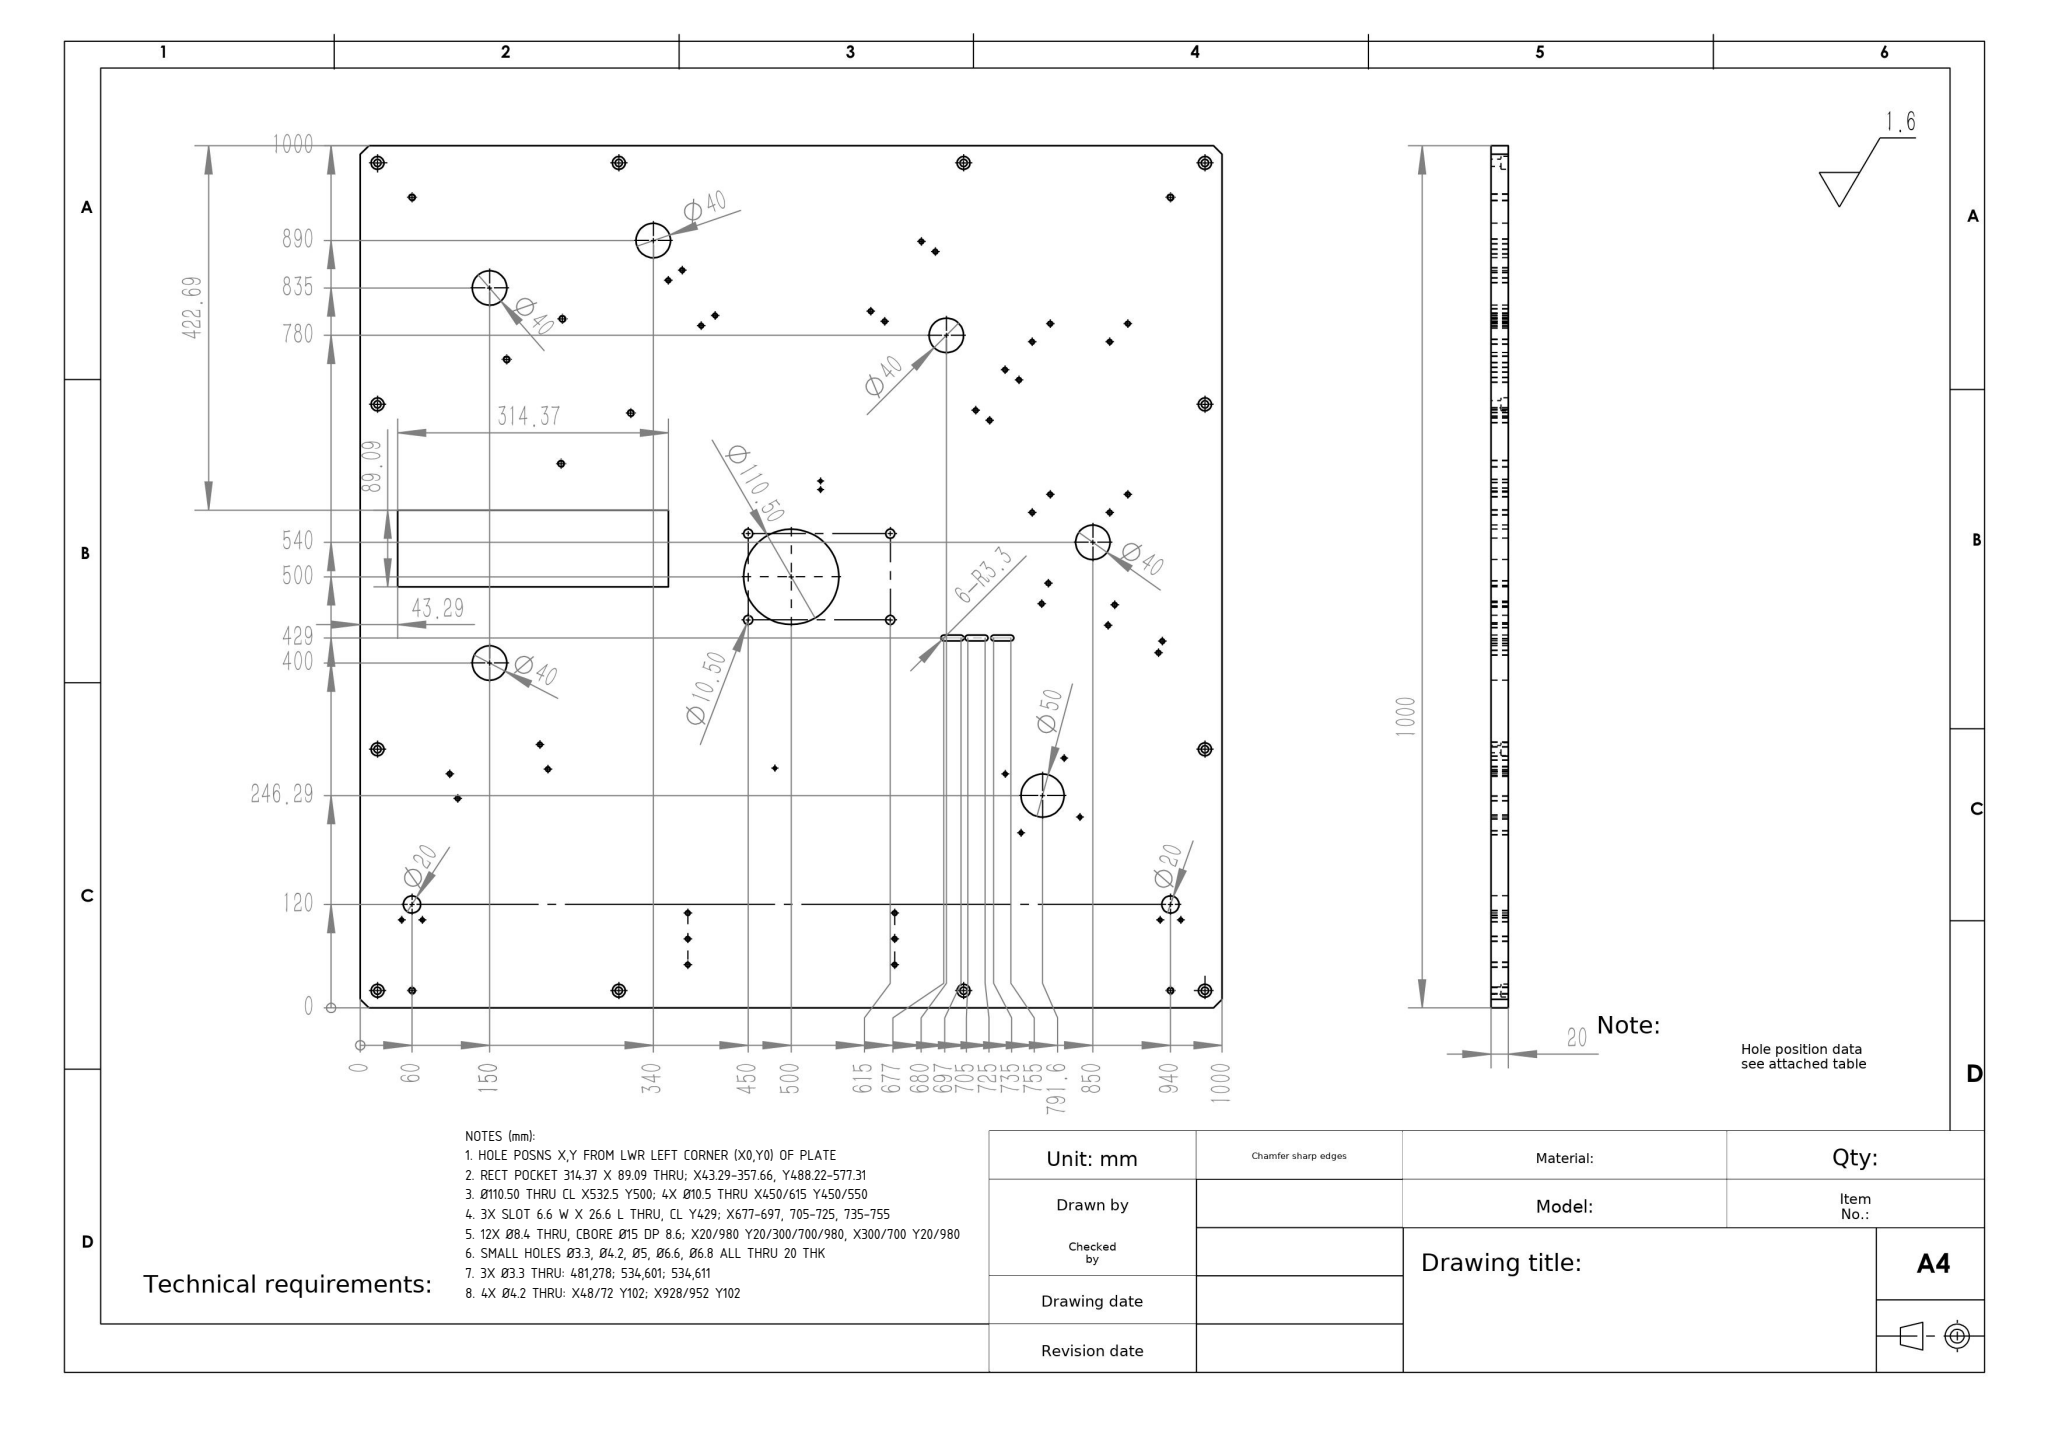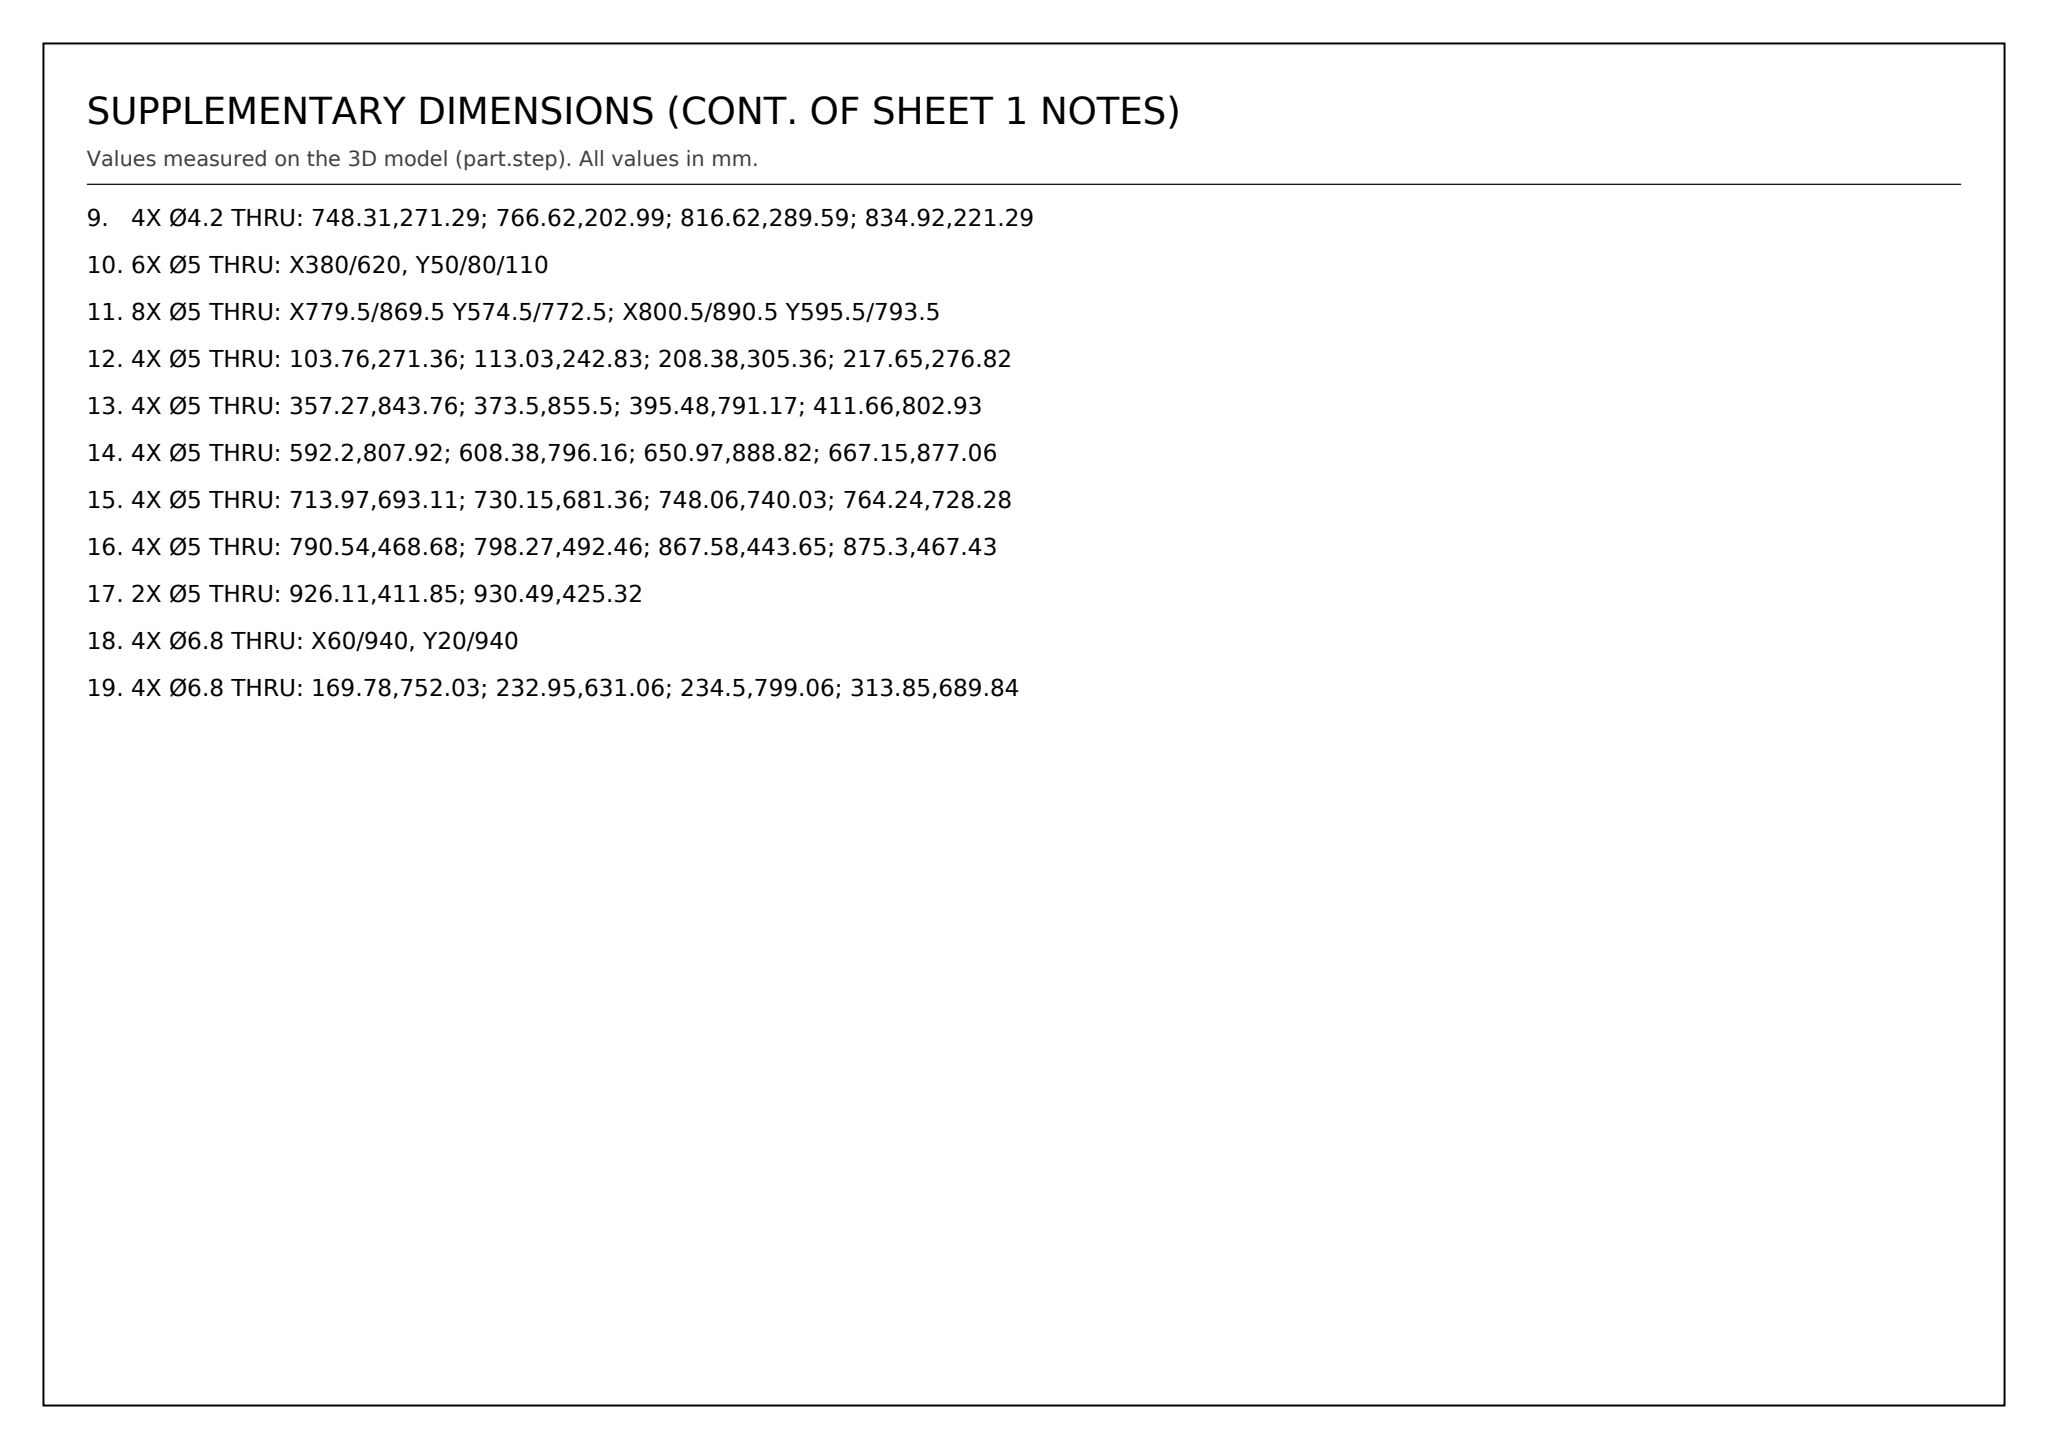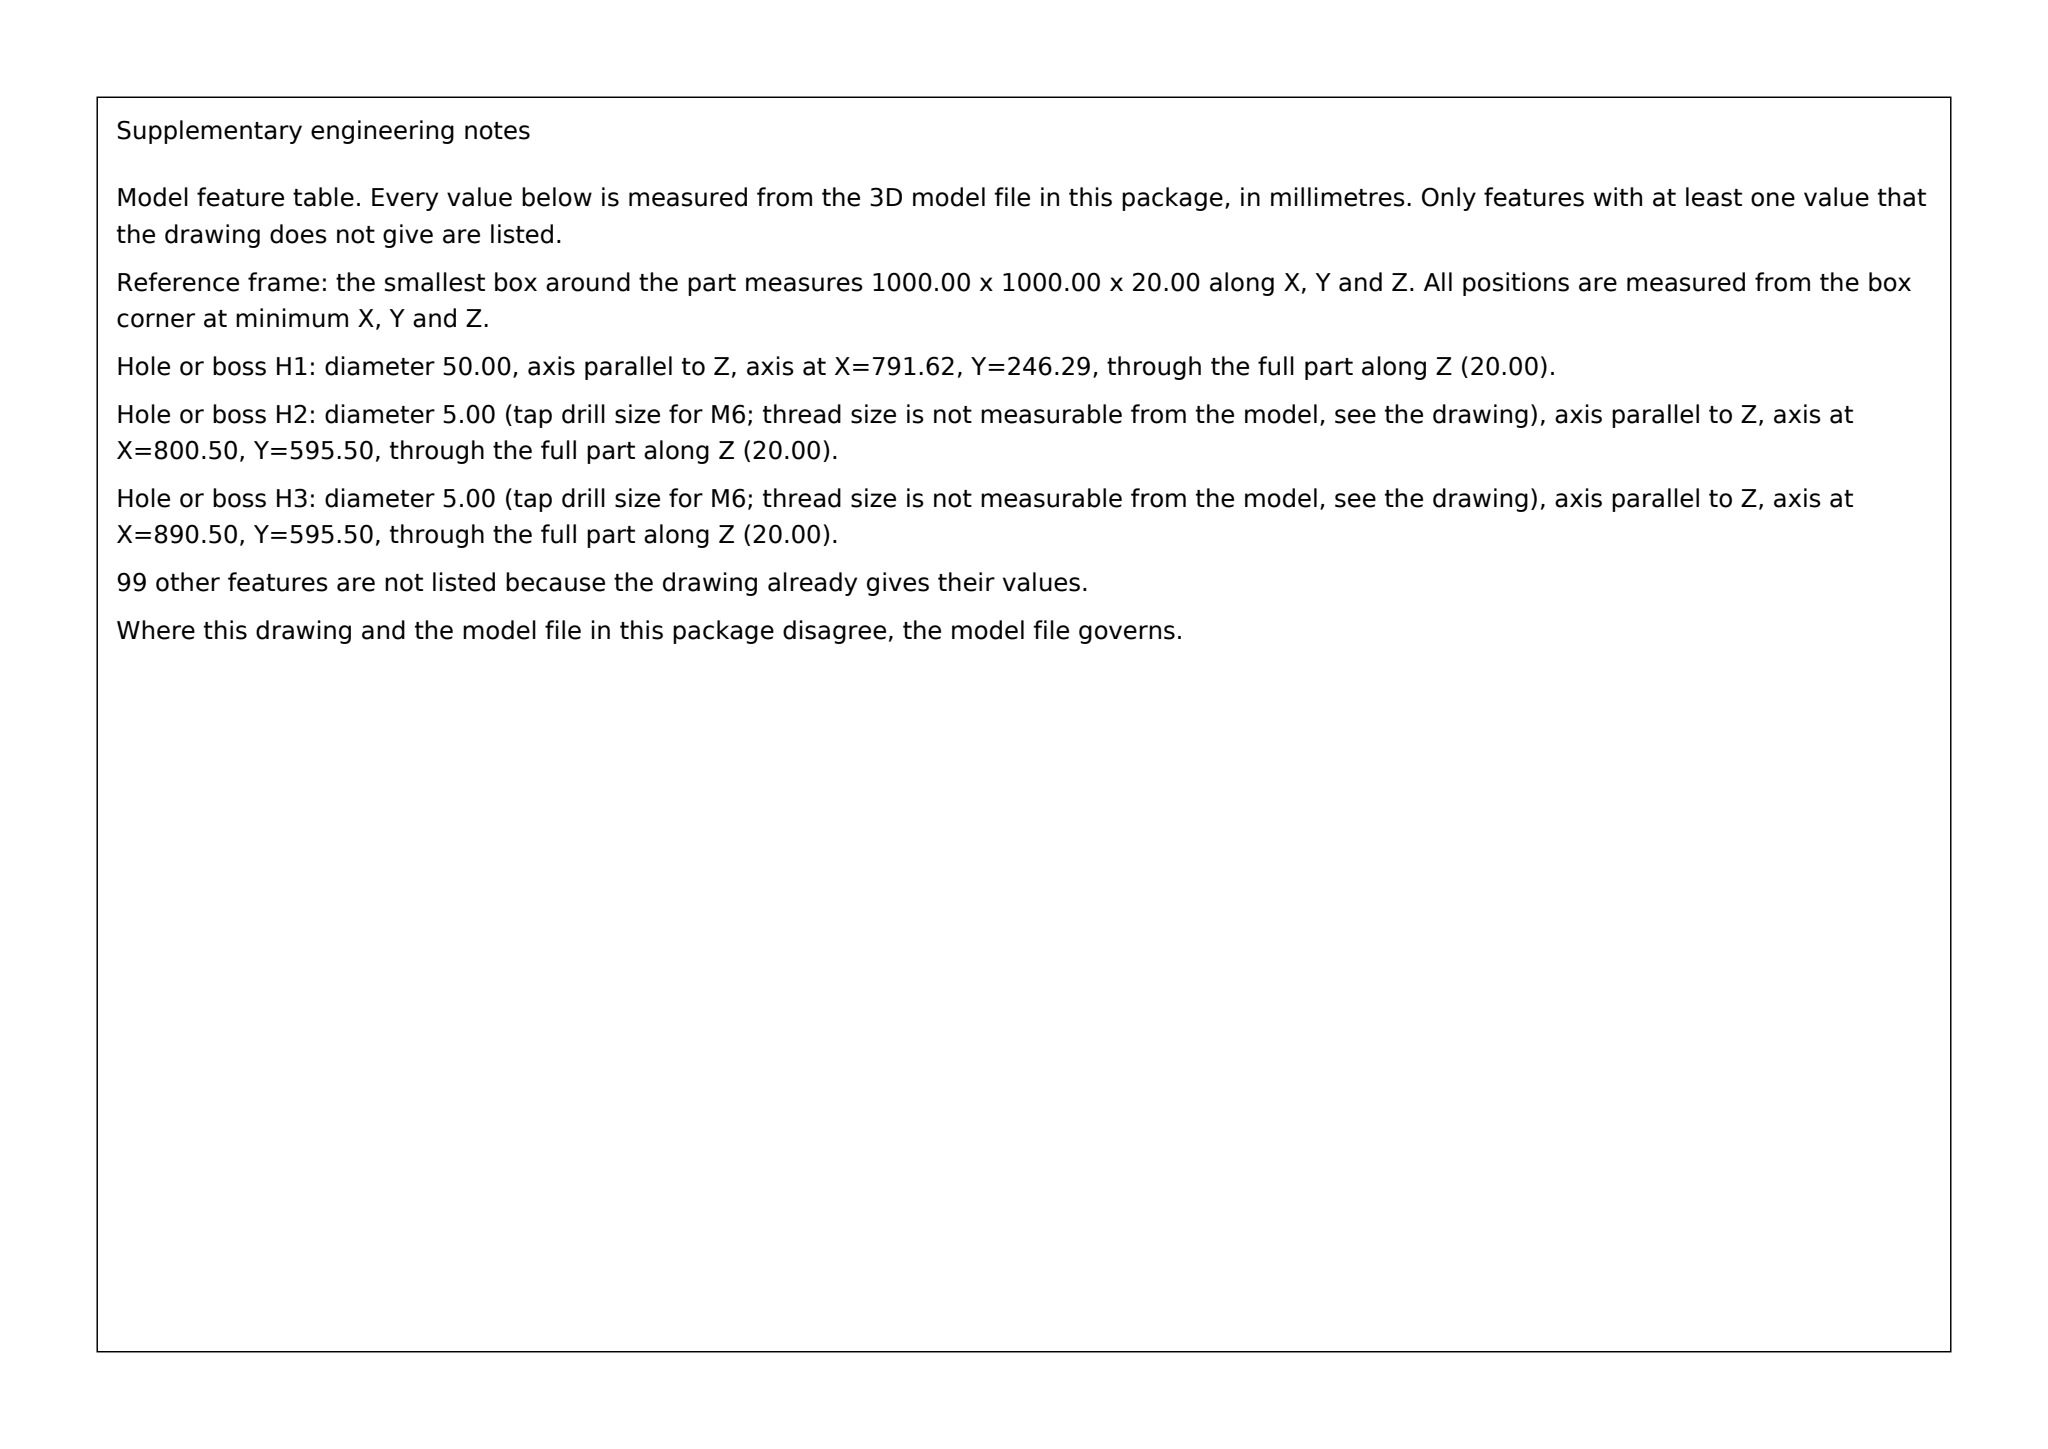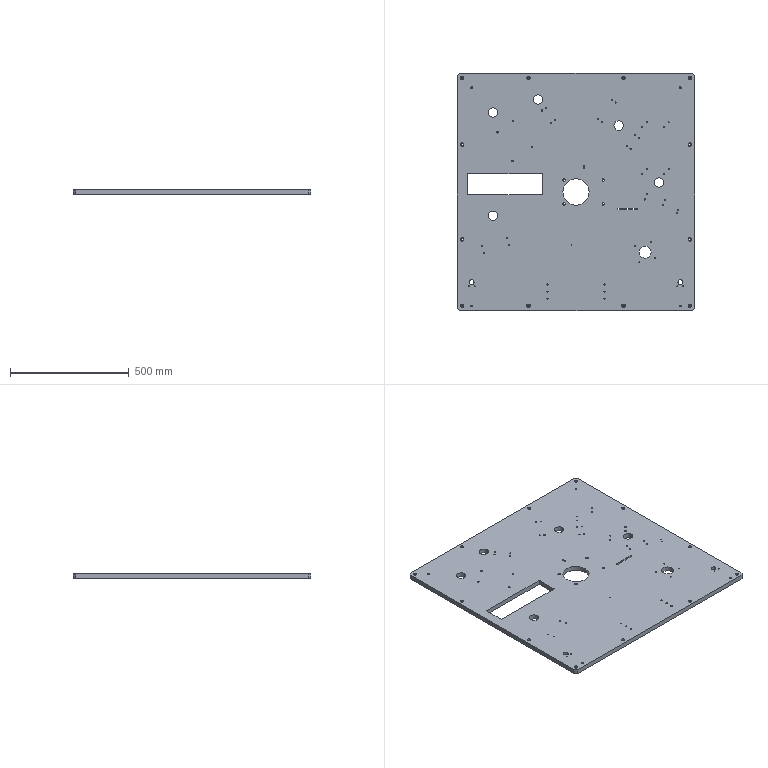Part | SolidWorks | mm | 1 solid | 225 faces | box 1000 x 1000 x 20 mm | volume 19001175 mm3 | cylinder 193 | plane 32 | commonest cylinder face diameters 5 x72 15 x24 8.4 x24 6.8 x16 4.2 x16 40 x10 6.6 x9 10.5 x8
Drawing notes:
HOLE POSNS X,Y FROM LWR LEFT CORNER (X0,Y0) OF PLATE | from the solid: origin_note: positions from min corner of 1000x1000x20 bbox
RECT POCKET 314.37 X 89.09 THRU; X43.29-357.66, Y488.22-577.31 | from the solid: planes x 43.29/357.66, y 488.22/577.31; z planes only 0/11.4/20 -> no pocket floor
Ø110.50 THRU CL X532.5 Y500; 4X Ø10.5 THRU X450/615 Y450/550 | from the solid: cyl Ø10.5 z L20 at (450,450)(450,550)(615,450)(615,550); pattern ctr 532.5,500
3X SLOT 6.6 W X 26.6 L THRU, CL Y429; X677-697, 705-725, 735-755 | from the solid: Ø6.6 z L20 at y429, x=677,697,705,725,735,755; y planes 425.7 & 432.3 (3 ea)
12X Ø8.4 THRU, CBORE Ø15 DP 8.6; X20/980 Y20/300/700/980, X300/700 Y20/980 | from the solid: Ø8.4 L11.4 + Ø15 L8.6 at (20,20)(20,300)(20,700)(20,980)(300,20)...(980,980); z-plane 11.4 count 12
SMALL HOLES Ø3.3, Ø4.2, Ø5, Ø6.6, Ø6.8 ALL THRU 20 THK | from the solid: cylinders dia 3.3/4.2/5.0/6.6/6.8, axis z, length 20 = full plate thk
3X Ø3.3 THRU: 481,278; 534,601; 534,611 | from the solid: [3.3,z,[481,278]],[3.3,z,[534,601]],[3.3,z,[534,611]]
4X Ø4.2 THRU: X48/72 Y102; X928/952 Y102 | from the solid: [4.2,z,[48,102]],[72,102],[928,102],[952,102]
4X Ø4.2 THRU: 748.31,271.29; 766.62,202.99; 816.62,289.59; 834.92,221.29 | from the solid: [4.2,z,[748.31,271.29]],[766.62,202.99],[816.62,289.59],[834.92,221.29]
6X Ø5 THRU: X380/620, Y50/80/110 | from the solid: [5,z,[380,50/80/110]],[5,z,[620,50/80/110]]
8X Ø5 THRU: X779.5/869.5 Y574.5/772.5; X800.5/890.5 Y595.5/793.5 | from the solid: [5,z,[779.5,574.5]],[779.5,772.5],[869.5,574.5],[869.5,772.5],[800.5,595.5],[800.5,793.5],[890.5,595.5],[890.5,793.5]
4X Ø5 THRU: 103.76,271.36; 113.03,242.83; 208.38,305.36; 217.65,276.82 | from the solid: [5,z,[103.76,271.36]],[113.03,242.83],[208.38,305.36],[217.65,276.82]
4X Ø5 THRU: 357.27,843.76; 373.5,855.5; 395.48,791.17; 411.66,802.93 | from the solid: [5,z,[357.27,843.76]],[373.5,855.5],[395.48,791.17],[411.66,802.93]
4X Ø5 THRU: 592.2,807.92; 608.38,796.16; 650.97,888.82; 667.15,877.06 | from the solid: [5,z,[592.2,807.92]],[608.38,796.16],[650.97,888.82],[667.15,877.06]
4X Ø5 THRU: 713.97,693.11; 730.15,681.36; 748.06,740.03; 764.24,728.28 | from the solid: [5,z,[713.97,693.11]],[730.15,681.36],[748.06,740.03],[764.24,728.28]
4X Ø5 THRU: 790.54,468.68; 798.27,492.46; 867.58,443.65; 875.3,467.43 | from the solid: [5,z,[790.54,468.68]],[798.27,492.46],[867.58,443.65],[875.3,467.43]
2X Ø5 THRU: 926.11,411.85; 930.49,425.32 | from the solid: [5,z,[926.11,411.85]],[5,z,[930.49,425.32]]
4X Ø6.8 THRU: X60/940, Y20/940 | from the solid: [6.8,z,[60,20]],[60,940],[940,20],[940,940]
4X Ø6.8 THRU: 169.78,752.03; 232.95,631.06; 234.5,799.06; 313.85,689.84 | from the solid: [6.8,z,[169.78,752.03]],[232.95,631.06],[234.5,799.06],[313.85,689.84]
build123d program:
from build123d import *

# Parameters (mm, degrees)
SKETCH1_W                                       = 1000
SKETCH1_H                                       = 1000
BOSS_EXTRUDE1_DEPTH                             = 20
CHAMFER1_SIZE                                   = 10
SKETCH2_R                                       = 55.25
CUT_EXTRUDE1_DEPTH                              = 708.39
M6_TAPPED_HOLE1_D                               = 5
SKETCH4_R                                       = 20
SKETCH4_R_2                                     = 25
CUT_EXTRUDE2_DEPTH                              = 708.39
M8_HEX_SOCKET_HEAD_CAP_SCREW_CBORE1_D           = 8.4
M8_HEX_SOCKET_HEAD_CAP_SCREW_CBORE1_CBORE_D     = 15
M8_HEX_SOCKET_HEAD_CAP_SCREW_CBORE1_CBORE_DEPTH = 8.6
F_6_5_6_5_DIAMETER_HOLE1_D                      = 6.5
F_10_5_10_5_DIAMETER_HOLE1_D                    = 10.5
M4_TAPPED_HOLE1_D                               = 3.3
M4_TAPPED_HOLE1_ON_FACE_2_D                     = 3.3
M8_TAPPED_HOLE1_D                               = 6.8
M5_TAPPED_HOLE1_D                               = 4.2
M8_TAPPED_HOLE2_D                               = 6.8
SKETCH13_R                                      = 10
CUT_EXTRUDE3_DEPTH                              = 708.39
CUT_EXTRUDE4_DEPTH                              = 708.39
SKETCH15_W                                      = 314.369
SKETCH15_H                                      = 89.088
CUT_EXTRUDE5_DEPTH                              = 469


with BuildPart() as part:
    # Sketch1 → Boss-Extrude1 (new body)
    with BuildSketch(Plane.XY):
        Rectangle(SKETCH1_W, SKETCH1_H)
    extrude(amount=BOSS_EXTRUDE1_DEPTH)

    # Chamfer1
    chamfer1_edges = [part.edges().sort_by_distance(p)[0] for p in [
        (500, -500, 10),
        (-500, -500, 10),
        (-500, 500, 10),
        (500, 500, 10),
    ]]
    chamfer(chamfer1_edges, length=CHAMFER1_SIZE)

    # Sketch2 → Cut-Extrude1 (cut, through all)
    with BuildSketch(Plane.XY.offset(20)):
        Circle(SKETCH2_R)
    extrude(amount=-CUT_EXTRUDE1_DEPTH, mode=Mode.SUBTRACT)

    # M6 Tapped Hole1 (through all)
    with Locations(Plane(origin=(-88.34, 302.93, 20), x_dir=(1, 0, 0), z_dir=(0, 0, 1))):
        with Locations((0, 0), (-16.18, -11.76), (-54.39, 40.83), (-38.16, 52.57), (239.31, 85.89), (255.49, 74.13), (180.54, 4.99), (196.72, -6.77), (336.4, -62.9), (352.58, -74.65), (302.31, -109.82), (318.49, -121.57), (386.61, -310.47), (378.88, -334.25), (463.64, -335.5), (455.92, -359.28), (518.83, -377.61), (514.45, -391.08), (367.84, -228.43), (388.84, -207.43), (388.84, -9.43), (367.84, -30.43), (478.84, -9.43), (457.84, -30.43), (478.84, -207.43), (457.84, -228.43), (-194.01, -526.11), (-203.28, -497.57), (-307.9, -531.57), (-298.63, -560.1), (208.34, -722.93), (208.34, -692.93), (208.34, -752.93), (-31.66, -752.93), (-31.66, -722.93), (-31.66, -692.93)):
            Hole(M6_TAPPED_HOLE1_D / 2)

    # Sketch4 → Cut-Extrude2 (cut, through all)
    with BuildSketch(Plane.XY.offset(20)):
        with Locations((-350, 335)):
            Circle(SKETCH4_R)
        with Locations((291.615, -253.708)):
            Circle(SKETCH4_R_2)
        with Locations((-350, -100)):
            Circle(SKETCH4_R)
        with Locations((350, 40)):
            Circle(SKETCH4_R)
        with Locations((180, 280)):
            Circle(SKETCH4_R)
        with Locations((-160, 390)):
            Circle(SKETCH4_R)
    extrude(amount=-CUT_EXTRUDE2_DEPTH, mode=Mode.SUBTRACT)

    # M8 Hex Socket Head Cap Screw CBORE1 (through all)
    with Locations(Plane(origin=(-480, 480, 20), x_dir=(1, 0, 0), z_dir=(0, 0, 1))):
        with Locations((0, 0), (280, 0), (680, 0), (960, 0), (960, -280), (960, -680), (960, -960), (680, -960), (280, -960), (0, -960), (0, -680), (0, -280)):
            CounterBoreHole(M8_HEX_SOCKET_HEAD_CAP_SCREW_CBORE1_D / 2, M8_HEX_SOCKET_HEAD_CAP_SCREW_CBORE1_CBORE_D / 2, M8_HEX_SOCKET_HEAD_CAP_SCREW_CBORE1_CBORE_DEPTH)

    # 6.5 _6.5_ Diameter Hole1 (through all)
    with Locations(Plane(origin=(241, -71, 20), x_dir=(1, 0, 0), z_dir=(0, 0, 1))):
        with Locations((0, 0), (-28, 0), (-56, 0)):
            Hole(F_6_5_6_5_DIAMETER_HOLE1_D / 2)

    # 10.5 _10.5_ Diameter Hole1 (through all)
    with Locations(Plane(origin=(-50, -50, 20), x_dir=(1, 0, 0), z_dir=(0, 0, 1))):
        with Locations((0, 0), (165, 0), (165, 100), (0, 100)):
            Hole(F_10_5_10_5_DIAMETER_HOLE1_D / 2)

    # M4 Tapped Hole1 (through all)
    with Locations(Plane(origin=(-19, -222, 20), x_dir=(1, 0, 0), z_dir=(0, 0, 1))):
        with Locations((0, 0)):
            Hole(M4_TAPPED_HOLE1_D / 2)

    # M4 Tapped Hole1 on face 2 (through all)
    with Locations(Plane(origin=(34, 111, 0), x_dir=(-1, 0, 0), z_dir=(0, 0, -1))):
        with Locations((0, 0), (0, -10)):
            Hole(M4_TAPPED_HOLE1_ON_FACE_2_D / 2)

    # M8 Tapped Hole1 (through all)
    with Locations(Plane(origin=(-267.05, 131.06, 20), x_dir=(1, 0, 0), z_dir=(0, 0, 1))):
        with Locations((0, 0), (-63.17, 120.97), (80.9, 58.78), (1.55, 168)):
            Hole(M8_TAPPED_HOLE1_D / 2)

    # M5 Tapped Hole1 (through all)
    with Locations(Plane(origin=(334.917, -278.708, 20), x_dir=(1, 0, 0), z_dir=(0, 0, 1))):
        with Locations((0, 0), (-68.301, -18.301), (-86.603, 50), (-18.301, 68.301), (-786.917, -119.292), (-762.917, -119.292), (117.083, -119.292), (93.083, -119.292)):
            Hole(M5_TAPPED_HOLE1_D / 2)

    # M8 Tapped Hole2 (through all)
    with Locations(Plane(origin=(-440, -480, 20), x_dir=(1, 0, 0), z_dir=(0, 0, 1))):
        with Locations((0, 0), (0, 920), (880, 920), (880, 0)):
            Hole(M8_TAPPED_HOLE2_D / 2)

    # Sketch13 → Cut-Extrude3 (cut, through all)
    with BuildSketch(Plane.XY.offset(20)):
        with Locations((-440, -380)):
            Circle(SKETCH13_R)
        with Locations(Location((440, -380, 0), (0, 0, 180))):
            Circle(SKETCH13_R)
    extrude(amount=-CUT_EXTRUDE3_DEPTH, mode=Mode.SUBTRACT)

    # Sketch14 → Cut-Extrude4 (cut, through all)
    with BuildSketch(Plane.XY.offset(20)):
        with BuildLine():
            Line((177, -67.7), (197, -67.7))
            ThreePointArc((197, -67.7), (200.3, -71), (197, -74.3))
            Line((197, -74.3), (177, -74.3))
            ThreePointArc((177, -74.3), (173.7, -71), (177, -67.7))
        make_face()
        with BuildLine():
            Line((205, -67.7), (225, -67.7))
            ThreePointArc((225, -67.7), (228.3, -71), (225, -74.3))
            Line((225, -74.3), (205, -74.3))
            ThreePointArc((205, -74.3), (201.7, -71), (205, -67.7))
        make_face()
        with BuildLine():
            Line((235, -67.7), (255, -67.7))
            ThreePointArc((255, -67.7), (258.3, -71), (255, -74.3))
            Line((255, -74.3), (235, -74.3))
            ThreePointArc((235, -74.3), (231.7, -71), (235, -67.7))
        make_face()
    extrude(amount=-CUT_EXTRUDE4_DEPTH, mode=Mode.SUBTRACT)

    # Sketch15 → Cut-Extrude5 (cut)
    with BuildSketch(Plane.XY.offset(20)):
        with Locations((-299.521, 32.768)):
            Rectangle(SKETCH15_W, SKETCH15_H)
    extrude(amount=-CUT_EXTRUDE5_DEPTH, mode=Mode.SUBTRACT)


solid = part.part